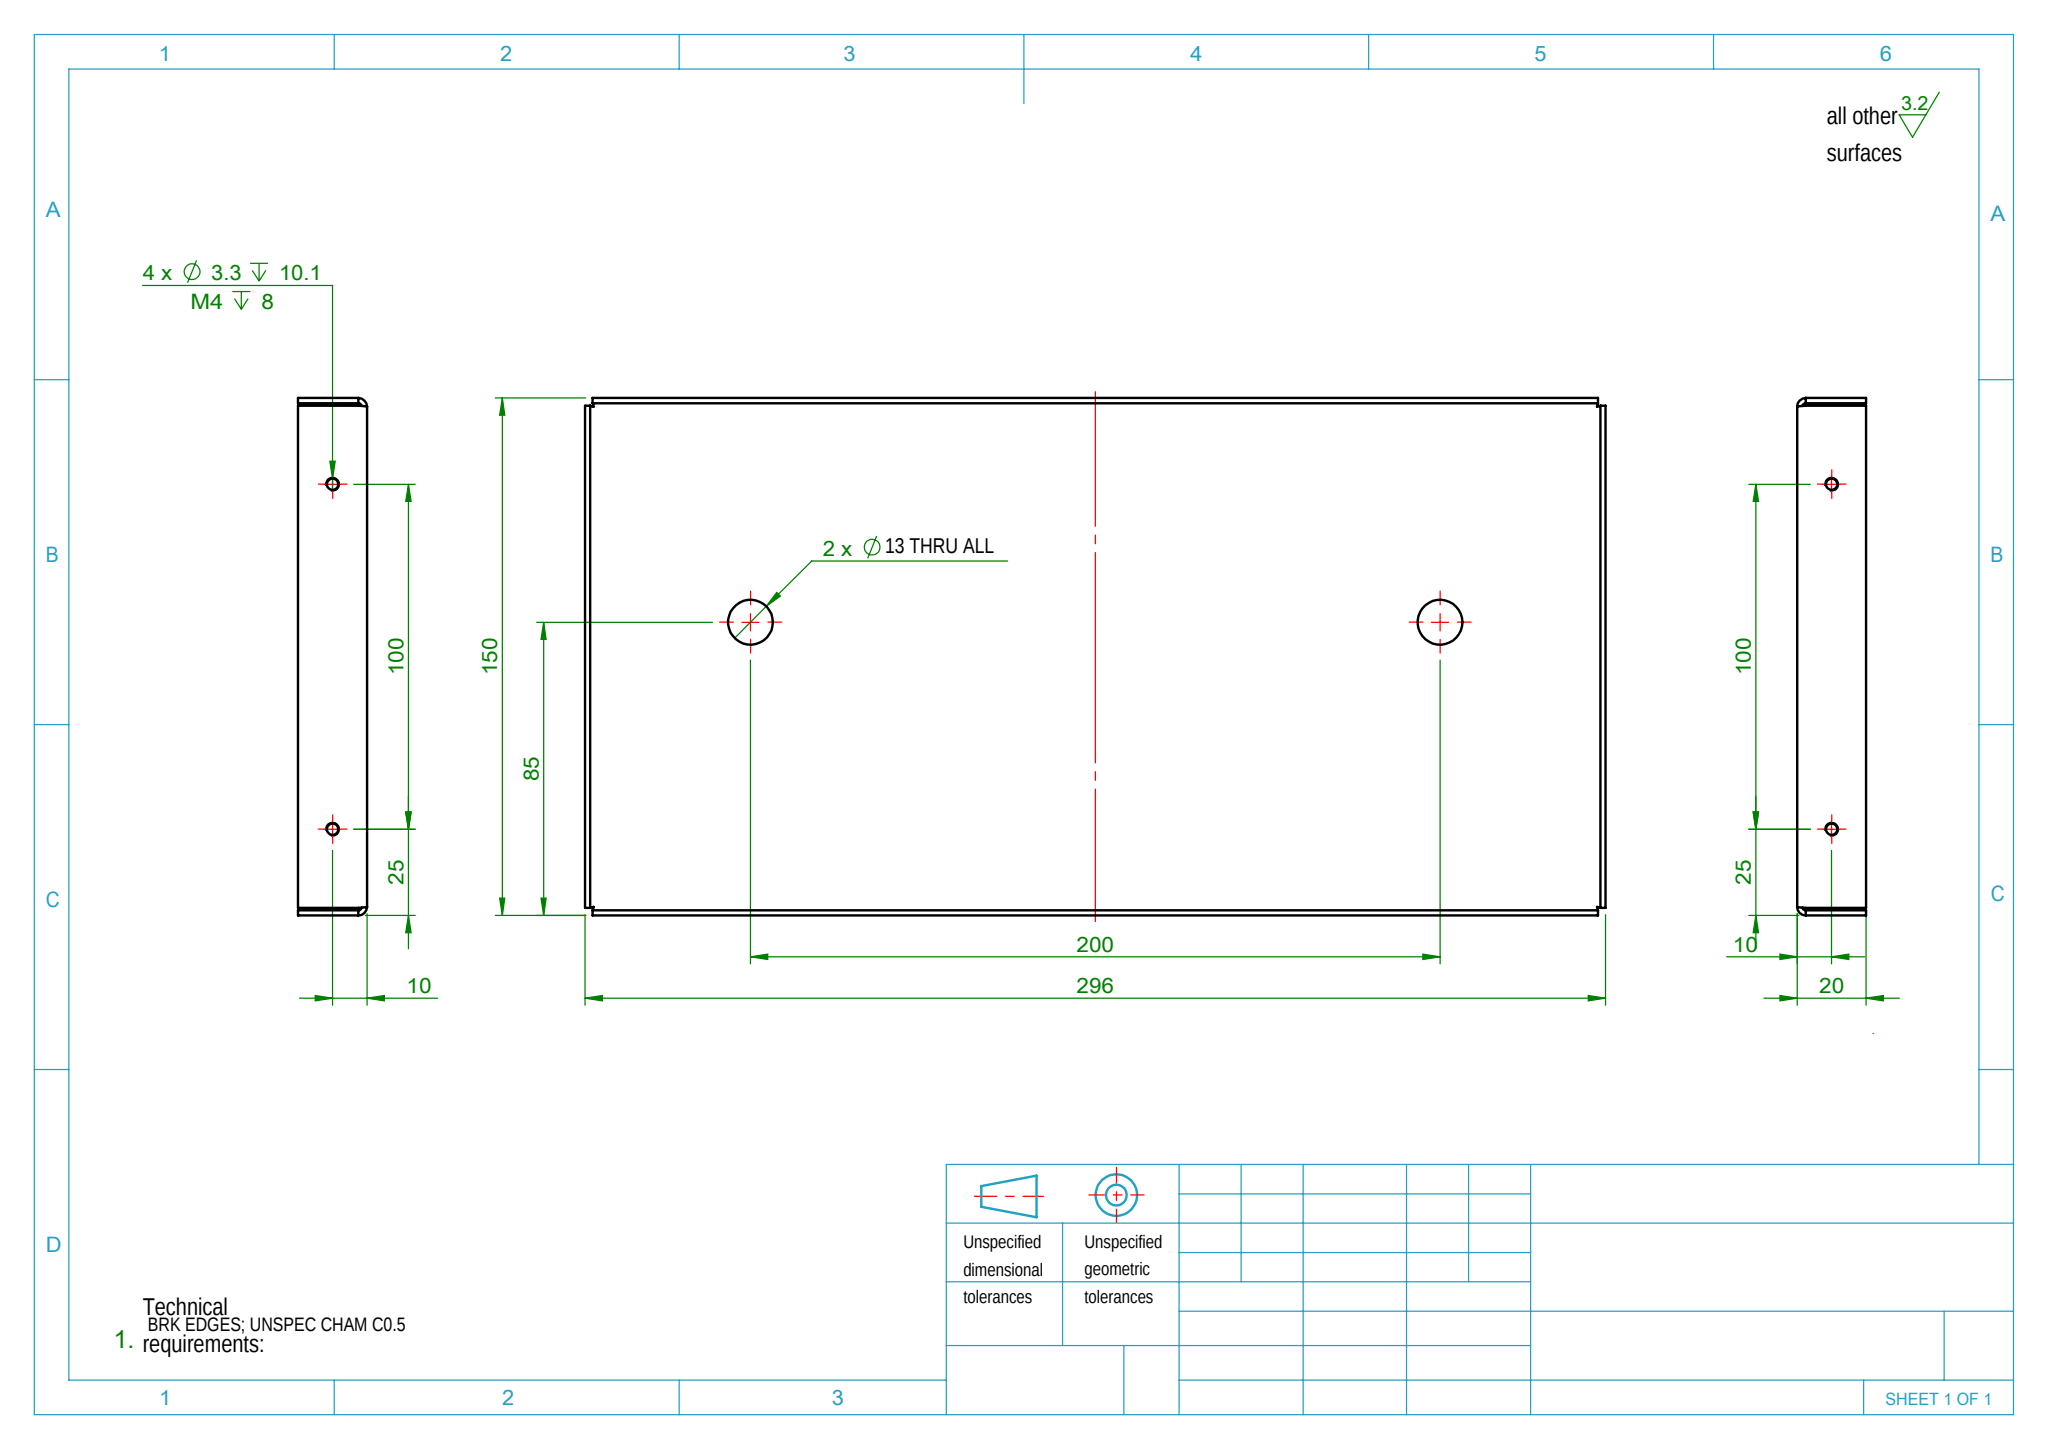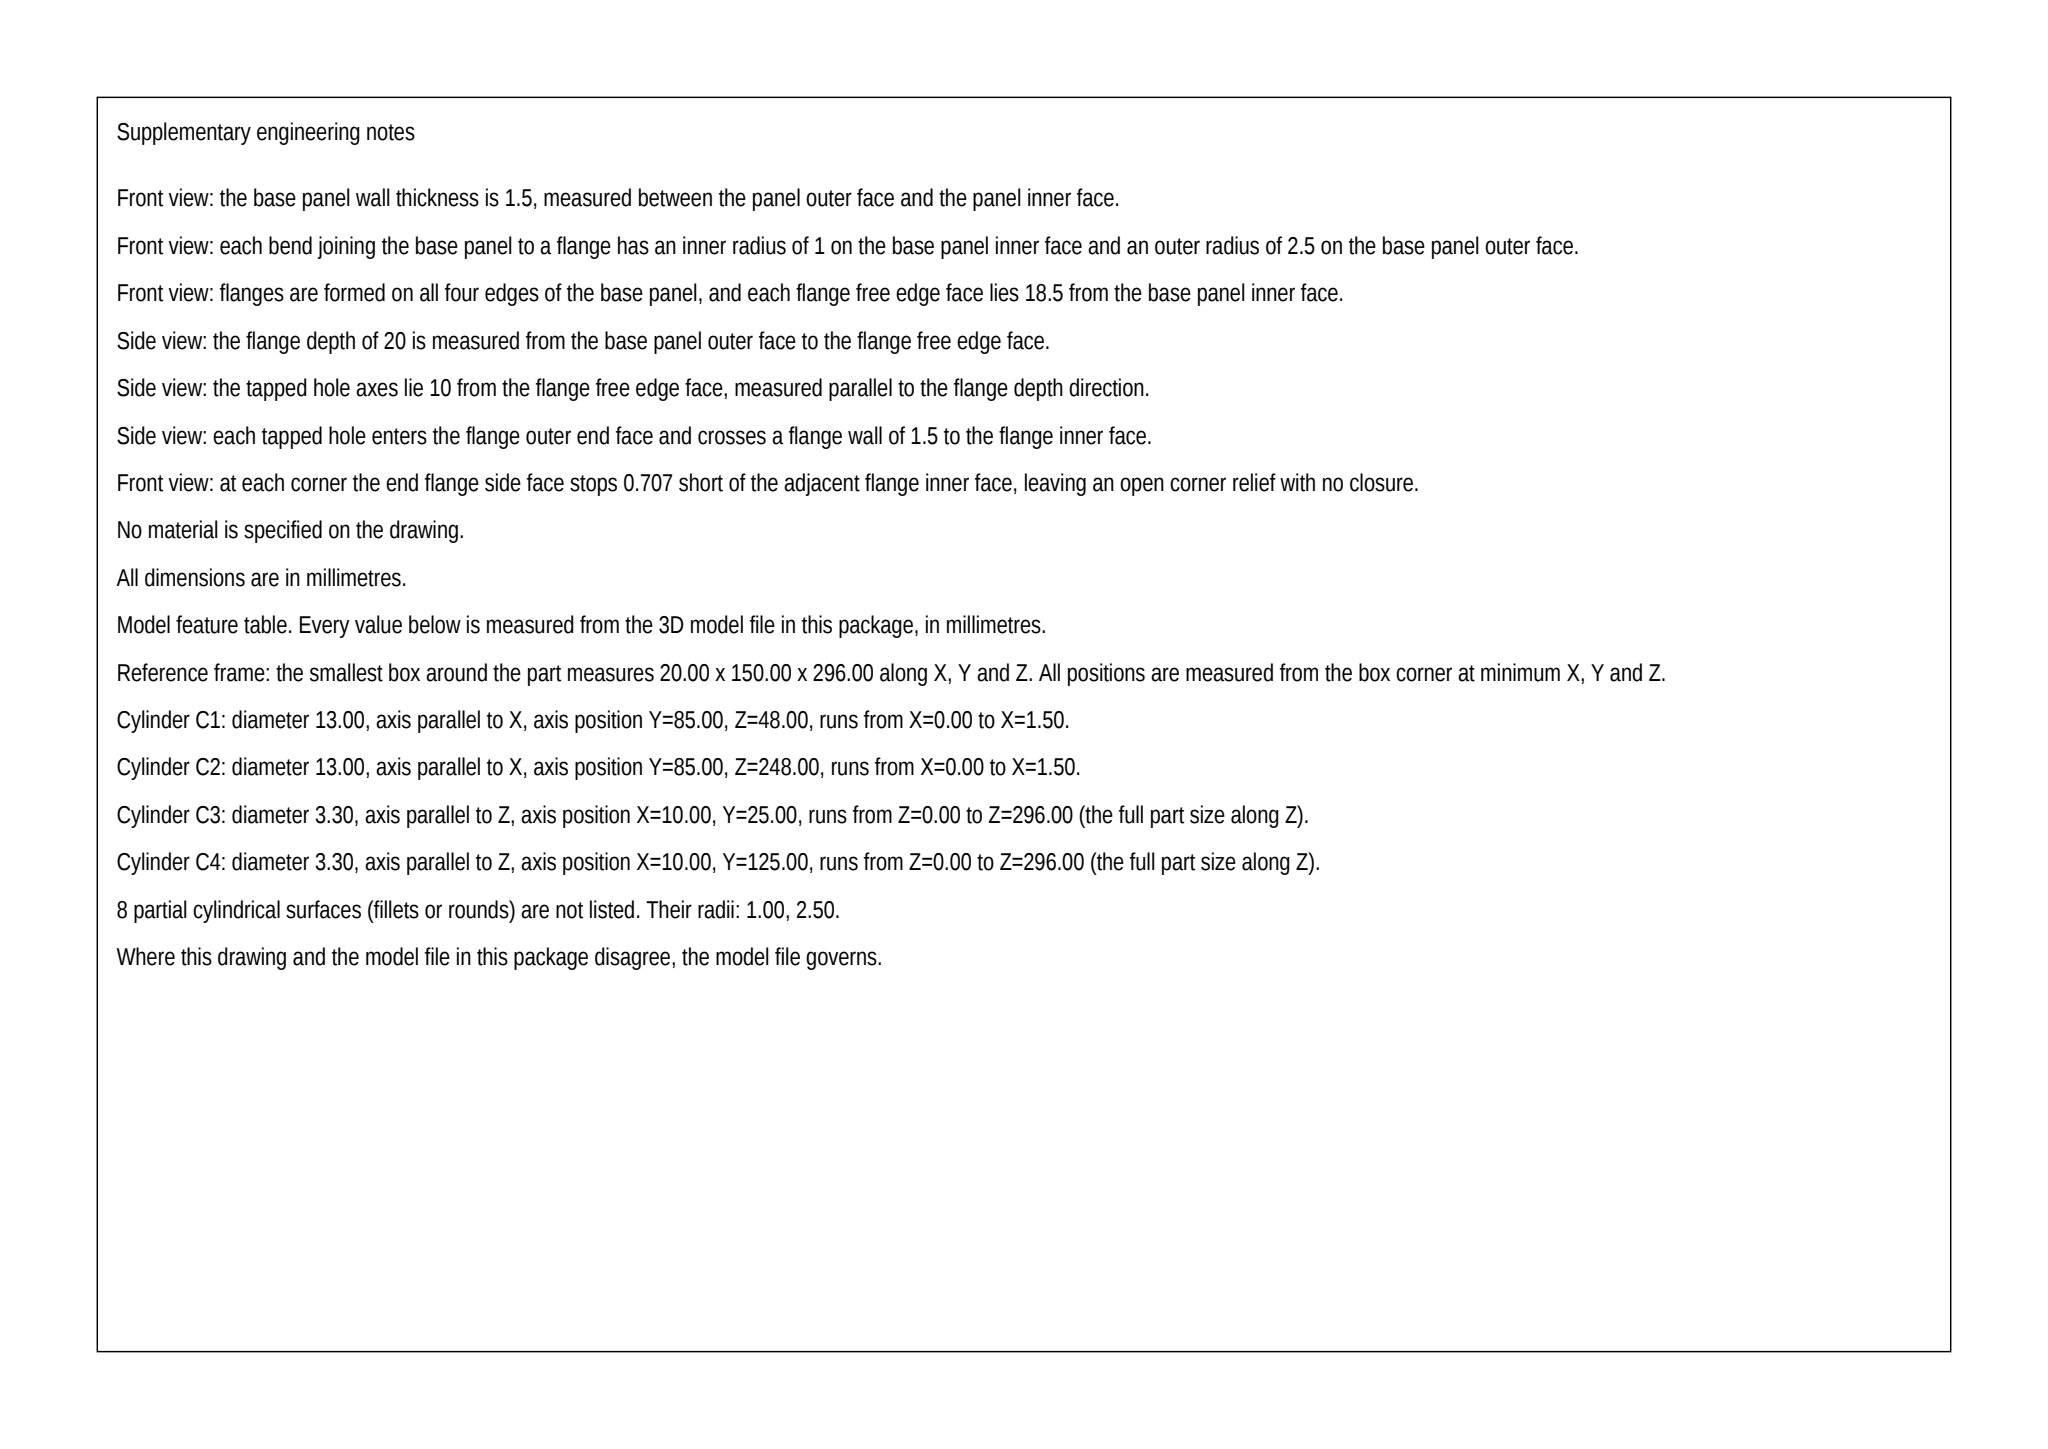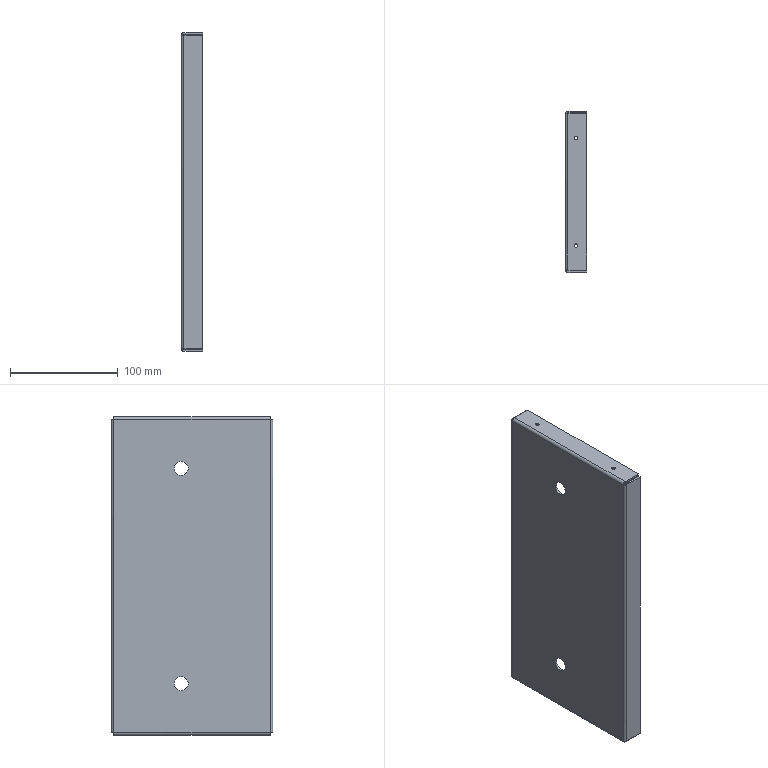Part | SolidWorks | mm | 1 solid | 50 faces | box 20 x 150 x 296 mm | volume 89395 mm3 | plane 22 | cylinder 20 | spline 8 | commonest cylinder face diameters 3.3 x8 13 x4 5 x4 2 x4
Drawing notes:
CORNER RELIEF: 0.7 GAP BTWN ADJ FLANGE ENDS, 4X CORNERS | from the solid: Flange inner faces y=1.52/148.52 & z=1.52/294.52; flange ends at y=2.22/147.81, z=2.22/293.81 => 0.7 setback gap at each of 4 corners
4X M4 THRU 1.5 THK FLANGE; TAP DRILL Ø3.3 THRU (NO 10.1/8 DEPTH) | from the solid: Cylinders dia 3.3, axis z, length 1.5 at (10.02,25.02) and (10.02,125.02); flange wall = planes z=0.02 to 1.52 = 1.5 thick